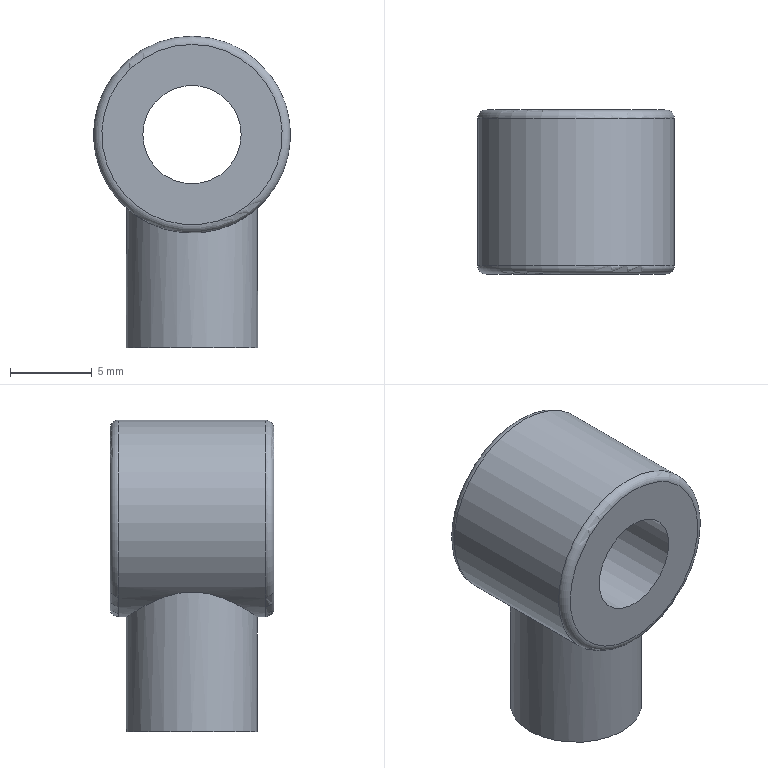Component | NX | PISTON_LINK | 1 solid | 10 faces | box 12 x 10 x 19 mm | volume 1057 mm3 | cylinder 4 | plane 4 | torus 2 | commonest cylinder face diameters 12 x1 6 x1 8 x1 5 x1
STEP:
#1=CARTESIAN_POINT('',(0.,0.,0.));
#2=DIRECTION('',(0.,0.,1.));
#3=DIRECTION('',(1.,0.,0.));
#4=AXIS2_PLACEMENT_3D('',#1,#2,#3);
#5=CARTESIAN_POINT('',(0.,-41.5,133.));
#6=VERTEX_POINT('',#5);
#7=CARTESIAN_POINT('',(0.,-41.5,127.));
#8=DIRECTION('',(0.,1.,0.));
#9=DIRECTION('',(0.,0.,1.));
#10=AXIS2_PLACEMENT_3D('',#7,#8,#9);
#11=CIRCLE('',#10,6.);
#12=CARTESIAN_POINT('',(0.,-32.,127.));
#13=DIRECTION('',(0.,-1.,0.));
#14=DIRECTION('',(0.,0.,1.));
#15=AXIS2_PLACEMENT_3D('',#12,#13,#14);
#16=CYLINDRICAL_SURFACE('',#15,6.);
#17=CARTESIAN_POINT('',(6.283,9.5));
#18=DIRECTION('',(-1.,0.));
#19=VECTOR('',#18,1.);
#20=LINE('',#17,#19);
#21=(GEOMETRIC_REPRESENTATION_CONTEXT(2)PARAMETRIC_REPRESENTATION_CONTEXT()REPRESENTATION_CONTEXT('',''));
#22=DEFINITIONAL_REPRESENTATION('',(#20),#21);
#23=PCURVE('',#16,#22);
#24=CARTESIAN_POINT('',(0.,-41.5,127.));
#25=DIRECTION('',(0.,-1.,0.));
#26=DIRECTION('',(0.,0.,1.));
#27=AXIS2_PLACEMENT_3D('',#24,#25,#26);
#28=TOROIDAL_SURFACE('',#27,5.5,0.5);
#29=CARTESIAN_POINT('',(6.283,6.283));
#30=DIRECTION('',(-1.,0.));
#31=VECTOR('',#30,1.);
#32=LINE('',#29,#31);
#33=(GEOMETRIC_REPRESENTATION_CONTEXT(2)PARAMETRIC_REPRESENTATION_CONTEXT()REPRESENTATION_CONTEXT('',''));
#34=DEFINITIONAL_REPRESENTATION('',(#32),#33);
#35=PCURVE('',#28,#34);
#36=SURFACE_CURVE('',#11,(#23,#35),.PCURVE_S1.);
#37=EDGE_CURVE('',#6,#6,#36,.T.);
#38=ORIENTED_EDGE('',*,*,#37,.T.);
#39=CARTESIAN_POINT('',(0.,-32.5,133.));
#40=VERTEX_POINT('',#39);
#41=CARTESIAN_POINT('',(0.,-32.5,133.));
#42=CARTESIAN_POINT('',(0.,-41.5,133.));
#43=B_SPLINE_CURVE_WITH_KNOTS('',1,(#41,#42),.UNSPECIFIED.,.F.,.F.,(2,2),(0.5,9.5),.PIECEWISE_BEZIER_KNOTS.);
#44=CARTESIAN_POINT('',(0.,0.));
#45=DIRECTION('',(0.,1.));
#46=VECTOR('',#45,1.);
#47=LINE('',#44,#46);
#48=(GEOMETRIC_REPRESENTATION_CONTEXT(2)PARAMETRIC_REPRESENTATION_CONTEXT()REPRESENTATION_CONTEXT('',''));
#49=DEFINITIONAL_REPRESENTATION('',(#47),#48);
#50=PCURVE('',#16,#49);
#51=CARTESIAN_POINT('',(6.283,0.));
#52=DIRECTION('',(0.,1.));
#53=VECTOR('',#52,1.);
#54=LINE('',#51,#53);
#55=(GEOMETRIC_REPRESENTATION_CONTEXT(2)PARAMETRIC_REPRESENTATION_CONTEXT()REPRESENTATION_CONTEXT('',''));
#56=DEFINITIONAL_REPRESENTATION('',(#54),#55);
#57=PCURVE('',#16,#56);
#58=SEAM_CURVE('',#43,(#50,#57),.PCURVE_S1.);
#59=EDGE_CURVE('',#40,#6,#58,.T.);
#60=ORIENTED_EDGE('',*,*,#59,.F.);
#61=CARTESIAN_POINT('',(0.,-32.5,127.));
#62=DIRECTION('',(0.,-1.,0.));
#63=DIRECTION('',(0.,0.,1.));
#64=AXIS2_PLACEMENT_3D('',#61,#62,#63);
#65=CIRCLE('',#64,6.);
#66=CARTESIAN_POINT('',(0.,0.5));
#67=DIRECTION('',(1.,0.));
#68=VECTOR('',#67,1.);
#69=LINE('',#66,#68);
#70=(GEOMETRIC_REPRESENTATION_CONTEXT(2)PARAMETRIC_REPRESENTATION_CONTEXT()REPRESENTATION_CONTEXT('',''));
#71=DEFINITIONAL_REPRESENTATION('',(#69),#70);
#72=PCURVE('',#16,#71);
#73=CARTESIAN_POINT('',(0.,-32.5,127.));
#74=DIRECTION('',(0.,-1.,0.));
#75=DIRECTION('',(0.,0.,1.));
#76=AXIS2_PLACEMENT_3D('',#73,#74,#75);
#77=TOROIDAL_SURFACE('',#76,5.5,0.5);
#78=CARTESIAN_POINT('',(0.,6.283));
#79=DIRECTION('',(1.,0.));
#80=VECTOR('',#79,1.);
#81=LINE('',#78,#80);
#82=(GEOMETRIC_REPRESENTATION_CONTEXT(2)PARAMETRIC_REPRESENTATION_CONTEXT()REPRESENTATION_CONTEXT('',''));
#83=DEFINITIONAL_REPRESENTATION('',(#81),#82);
#84=PCURVE('',#77,#83);
#85=SURFACE_CURVE('',#65,(#72,#84),.PCURVE_S1.);
#86=EDGE_CURVE('',#40,#40,#85,.T.);
#87=ORIENTED_EDGE('',*,*,#86,.T.);
#88=ORIENTED_EDGE('',*,*,#59,.T.);
#89=EDGE_LOOP('',(#38,#60,#87,#88));
#90=FACE_BOUND('',#89,.T.);
#91=CARTESIAN_POINT('',(0.,-33.,121.));
#92=VERTEX_POINT('',#91);
#93=CARTESIAN_POINT('',(1.094,-33.,121.));
#94=CARTESIAN_POINT('',(-1.094,-33.,121.));
#95=CARTESIAN_POINT('',(-2.121,-33.461,121.329));
#96=CARTESIAN_POINT('',(-3.548,-34.894,122.094));
#97=CARTESIAN_POINT('',(-3.998,-35.907,122.526));
#98=CARTESIAN_POINT('',(-4.002,-38.077,122.53));
#99=CARTESIAN_POINT('',(-3.557,-39.094,122.1));
#100=CARTESIAN_POINT('',(-2.124,-40.539,121.33));
#101=CARTESIAN_POINT('',(-1.087,-40.998,121.002));
#102=CARTESIAN_POINT('',(1.069,-41.002,120.998));
#103=CARTESIAN_POINT('',(2.12,-40.54,121.329));
#104=CARTESIAN_POINT('',(3.55,-39.103,122.095));
#105=CARTESIAN_POINT('',(4.,-38.095,122.527));
#106=CARTESIAN_POINT('',(4.,-35.908,122.528));
#107=CARTESIAN_POINT('',(3.55,-34.897,122.095));
#108=CARTESIAN_POINT('',(2.122,-33.462,121.33));
#109=CARTESIAN_POINT('',(1.094,-33.,121.));
#110=CARTESIAN_POINT('',(-1.094,-33.,121.));
#111=B_SPLINE_CURVE_WITH_KNOTS('',3,(#93,#94,#95,#96,#97,#98,#99,#100,#101,#102,#103,#104,#105,#106,#107,#108,#109,#110),.UNSPECIFIED.,.T.,.F.,(2,2,2,2,2,2,2,2,2,2,2),(-0.125,0.,0.125,0.25,0.375,0.5,0.625,0.75,0.875,1.,1.125),.UNSPECIFIED.);
#112=CARTESIAN_POINT('',(3.142,1.));
#113=CARTESIAN_POINT('',(3.108,1.));
#114=CARTESIAN_POINT('',(3.043,1.03));
#115=CARTESIAN_POINT('',(2.947,1.16));
#116=CARTESIAN_POINT('',(2.855,1.367));
#117=CARTESIAN_POINT('',(2.767,1.642));
#118=CARTESIAN_POINT('',(2.686,1.98));
#119=CARTESIAN_POINT('',(2.612,2.371));
#120=CARTESIAN_POINT('',(2.546,2.818));
#121=CARTESIAN_POINT('',(2.491,3.311));
#122=CARTESIAN_POINT('',(2.447,3.843));
#123=CARTESIAN_POINT('',(2.419,4.405));
#124=CARTESIAN_POINT('',(2.408,4.992));
#125=CARTESIAN_POINT('',(2.418,5.58));
#126=CARTESIAN_POINT('',(2.446,6.143));
#127=CARTESIAN_POINT('',(2.489,6.676));
#128=CARTESIAN_POINT('',(2.545,7.172));
#129=CARTESIAN_POINT('',(2.611,7.621));
#130=CARTESIAN_POINT('',(2.685,8.016));
#131=CARTESIAN_POINT('',(2.767,8.355));
#132=CARTESIAN_POINT('',(2.855,8.632));
#133=CARTESIAN_POINT('',(2.947,8.838));
#134=CARTESIAN_POINT('',(3.043,8.969));
#135=CARTESIAN_POINT('',(3.14,9.015));
#136=CARTESIAN_POINT('',(3.238,8.971));
#137=CARTESIAN_POINT('',(3.334,8.841));
#138=CARTESIAN_POINT('',(3.427,8.635));
#139=CARTESIAN_POINT('',(3.515,8.358));
#140=CARTESIAN_POINT('',(3.597,8.02));
#141=CARTESIAN_POINT('',(3.671,7.628));
#142=CARTESIAN_POINT('',(3.737,7.181));
#143=CARTESIAN_POINT('',(3.793,6.688));
#144=CARTESIAN_POINT('',(3.836,6.156));
#145=CARTESIAN_POINT('',(3.864,5.593));
#146=CARTESIAN_POINT('',(3.875,5.002));
#147=CARTESIAN_POINT('',(3.864,4.41));
#148=CARTESIAN_POINT('',(3.836,3.846));
#149=CARTESIAN_POINT('',(3.793,3.313));
#150=CARTESIAN_POINT('',(3.737,2.82));
#151=CARTESIAN_POINT('',(3.671,2.373));
#152=CARTESIAN_POINT('',(3.597,1.981));
#153=CARTESIAN_POINT('',(3.516,1.643));
#154=CARTESIAN_POINT('',(3.428,1.367));
#155=CARTESIAN_POINT('',(3.336,1.16));
#156=CARTESIAN_POINT('',(3.24,1.031));
#157=CARTESIAN_POINT('',(3.175,1.));
#158=CARTESIAN_POINT('',(3.142,1.));
#159=B_SPLINE_CURVE_WITH_KNOTS('',3,(#112,#113,#114,#115,#116,#117,#118,#119,#120,#121,#122,#123,#124,#125,#126,#127,#128,#129,#130,#131,#132,#133,#134,#135,#136,#137,#138,#139,#140,#141,#142,#143,#144,#145,#146,#147,#148,#149,#150,#151,#152,#153,#154,#155,#156,#157,#158),.UNSPECIFIED.,.T.,.F.,(4,1,1,1,1,1,1,1,1,1,1,1,1,1,1,1,1,1,1,1,1,1,1,1,1,1,1,1,1,1,1,1,1,1,1,1,1,1,1,1,1,1,1,1,4),(0.,0.02273,0.04545,0.06818,0.09091,0.1136,0.1364,0.1591,0.1818,0.2045,0.2273,0.25,0.2727,0.2955,0.3182,0.3409,0.3636,0.3864,0.4091,0.4318,0.4545,0.4773,0.5,0.5227,0.5455,0.5682,0.5909,0.6136,0.6364,0.6591,0.6818,0.7045,0.7273,0.75,0.7727,0.7955,0.8182,0.8409,0.8636,0.8864,0.9091,0.9318,0.9545,0.9773,1.),.QUASI_UNIFORM_KNOTS.);
#160=(GEOMETRIC_REPRESENTATION_CONTEXT(2)PARAMETRIC_REPRESENTATION_CONTEXT()REPRESENTATION_CONTEXT('',''));
#161=DEFINITIONAL_REPRESENTATION('',(#159),#160);
#162=PCURVE('',#16,#161);
#163=CARTESIAN_POINT('',(0.,-37.,114.));
#164=DIRECTION('',(0.,0.,1.));
#165=DIRECTION('',(0.,1.,0.));
#166=AXIS2_PLACEMENT_3D('',#163,#164,#165);
#167=CYLINDRICAL_SURFACE('',#166,4.);
#168=CARTESIAN_POINT('',(0.,7.));
#169=CARTESIAN_POINT('',(0.04968,7.));
#170=CARTESIAN_POINT('',(0.1481,7.022));
#171=CARTESIAN_POINT('',(0.2934,7.11));
#172=CARTESIAN_POINT('',(0.437,7.243));
#173=CARTESIAN_POINT('',(0.5788,7.412));
#174=CARTESIAN_POINT('',(0.7187,7.606));
#175=CARTESIAN_POINT('',(0.8564,7.817));
#176=CARTESIAN_POINT('',(0.9956,8.029));
#177=CARTESIAN_POINT('',(1.136,8.224));
#178=CARTESIAN_POINT('',(1.278,8.387));
#179=CARTESIAN_POINT('',(1.422,8.498));
#180=CARTESIAN_POINT('',(1.569,8.542));
#181=CARTESIAN_POINT('',(1.716,8.5));
#182=CARTESIAN_POINT('',(1.86,8.39));
#183=CARTESIAN_POINT('',(2.002,8.229));
#184=CARTESIAN_POINT('',(2.143,8.033));
#185=CARTESIAN_POINT('',(2.283,7.821));
#186=CARTESIAN_POINT('',(2.421,7.609));
#187=CARTESIAN_POINT('',(2.562,7.414));
#188=CARTESIAN_POINT('',(2.704,7.244));
#189=CARTESIAN_POINT('',(2.848,7.111));
#190=CARTESIAN_POINT('',(2.993,7.022));
#191=CARTESIAN_POINT('',(3.139,6.989));
#192=CARTESIAN_POINT('',(3.286,7.021));
#193=CARTESIAN_POINT('',(3.432,7.109));
#194=CARTESIAN_POINT('',(3.576,7.242));
#195=CARTESIAN_POINT('',(3.719,7.412));
#196=CARTESIAN_POINT('',(3.86,7.606));
#197=CARTESIAN_POINT('',(3.998,7.817));
#198=CARTESIAN_POINT('',(4.138,8.03));
#199=CARTESIAN_POINT('',(4.278,8.225));
#200=CARTESIAN_POINT('',(4.42,8.388));
#201=CARTESIAN_POINT('',(4.564,8.499));
#202=CARTESIAN_POINT('',(4.712,8.542));
#203=CARTESIAN_POINT('',(4.86,8.499));
#204=CARTESIAN_POINT('',(5.004,8.388));
#205=CARTESIAN_POINT('',(5.146,8.226));
#206=CARTESIAN_POINT('',(5.287,8.03));
#207=CARTESIAN_POINT('',(5.426,7.818));
#208=CARTESIAN_POINT('',(5.564,7.607));
#209=CARTESIAN_POINT('',(5.704,7.413));
#210=CARTESIAN_POINT('',(5.846,7.243));
#211=CARTESIAN_POINT('',(5.99,7.11));
#212=CARTESIAN_POINT('',(6.135,7.022));
#213=CARTESIAN_POINT('',(6.234,7.));
#214=CARTESIAN_POINT('',(6.283,7.));
#215=B_SPLINE_CURVE_WITH_KNOTS('',3,(#168,#169,#170,#171,#172,#173,#174,#175,#176,#177,#178,#179,#180,#181,#182,#183,#184,#185,#186,#187,#188,#189,#190,#191,#192,#193,#194,#195,#196,#197,#198,#199,#200,#201,#202,#203,#204,#205,#206,#207,#208,#209,#210,#211,#212,#213,#214),.UNSPECIFIED.,.F.,.F.,(4,1,1,1,1,1,1,1,1,1,1,1,1,1,1,1,1,1,1,1,1,1,1,1,1,1,1,1,1,1,1,1,1,1,1,1,1,1,1,1,1,1,1,1,4),(0.,0.02273,0.04545,0.06818,0.09091,0.1136,0.1364,0.1591,0.1818,0.2045,0.2273,0.25,0.2727,0.2955,0.3182,0.3409,0.3636,0.3864,0.4091,0.4318,0.4545,0.4773,0.5,0.5227,0.5455,0.5682,0.5909,0.6136,0.6364,0.6591,0.6818,0.7045,0.7273,0.75,0.7727,0.7955,0.8182,0.8409,0.8636,0.8864,0.9091,0.9318,0.9545,0.9773,1.),.QUASI_UNIFORM_KNOTS.);
#216=(GEOMETRIC_REPRESENTATION_CONTEXT(2)PARAMETRIC_REPRESENTATION_CONTEXT()REPRESENTATION_CONTEXT('',''));
#217=DEFINITIONAL_REPRESENTATION('',(#215),#216);
#218=PCURVE('',#167,#217);
#219=SURFACE_CURVE('',#111,(#162,#218),.PCURVE_S1.);
#220=EDGE_CURVE('',#92,#92,#219,.T.);
#221=ORIENTED_EDGE('',*,*,#220,.T.);
#222=EDGE_LOOP('',(#221));
#223=FACE_BOUND('',#222,.T.);
#224=ADVANCED_FACE('',(#90,#223),#16,.T.);
#225=CARTESIAN_POINT('',(-3.,-32.,127.));
#226=VERTEX_POINT('',#225);
#227=CARTESIAN_POINT('',(0.,-32.,127.));
#228=DIRECTION('',(0.,-1.,0.));
#229=DIRECTION('',(-1.,0.,0.));
#230=AXIS2_PLACEMENT_3D('',#227,#228,#229);
#231=CIRCLE('',#230,3.);
#232=CARTESIAN_POINT('',(0.,-32.,127.));
#233=DIRECTION('',(0.,-1.,0.));
#234=DIRECTION('',(0.,0.,1.));
#235=AXIS2_PLACEMENT_3D('',#232,#233,#234);
#236=CYLINDRICAL_SURFACE('',#235,3.);
#237=CARTESIAN_POINT('',(1.571,0.));
#238=DIRECTION('',(1.,0.));
#239=VECTOR('',#238,1.);
#240=LINE('',#237,#239);
#241=(GEOMETRIC_REPRESENTATION_CONTEXT(2)PARAMETRIC_REPRESENTATION_CONTEXT()REPRESENTATION_CONTEXT('',''));
#242=DEFINITIONAL_REPRESENTATION('',(#240),#241);
#243=PCURVE('',#236,#242);
#244=CARTESIAN_POINT('',(0.,-32.,127.));
#245=DIRECTION('',(0.,-1.,0.));
#246=DIRECTION('',(0.,0.,1.));
#247=AXIS2_PLACEMENT_3D('',#244,#245,#246);
#248=PLANE('',#247);
#249=CARTESIAN_POINT('',(0.,0.));
#250=DIRECTION('',(0.,1.));
#251=AXIS2_PLACEMENT_2D('',#249,#250);
#252=CIRCLE('',#251,3.);
#253=(GEOMETRIC_REPRESENTATION_CONTEXT(2)PARAMETRIC_REPRESENTATION_CONTEXT()REPRESENTATION_CONTEXT('',''));
#254=DEFINITIONAL_REPRESENTATION('',(#252),#253);
#255=PCURVE('',#248,#254);
#256=SURFACE_CURVE('',#231,(#243,#255),.PCURVE_S1.);
#257=EDGE_CURVE('',#226,#226,#256,.T.);
#258=ORIENTED_EDGE('',*,*,#257,.T.);
#259=CARTESIAN_POINT('',(-3.,-42.,127.));
#260=VERTEX_POINT('',#259);
#261=CARTESIAN_POINT('',(-3.,-32.,127.));
#262=CARTESIAN_POINT('',(-3.,-42.,127.));
#263=B_SPLINE_CURVE_WITH_KNOTS('',1,(#261,#262),.UNSPECIFIED.,.F.,.F.,(2,2),(0.,10.),.PIECEWISE_BEZIER_KNOTS.);
#264=CARTESIAN_POINT('',(7.854,0.));
#265=DIRECTION('',(0.,1.));
#266=VECTOR('',#265,1.);
#267=LINE('',#264,#266);
#268=(GEOMETRIC_REPRESENTATION_CONTEXT(2)PARAMETRIC_REPRESENTATION_CONTEXT()REPRESENTATION_CONTEXT('',''));
#269=DEFINITIONAL_REPRESENTATION('',(#267),#268);
#270=PCURVE('',#236,#269);
#271=CARTESIAN_POINT('',(1.571,0.));
#272=DIRECTION('',(0.,1.));
#273=VECTOR('',#272,1.);
#274=LINE('',#271,#273);
#275=(GEOMETRIC_REPRESENTATION_CONTEXT(2)PARAMETRIC_REPRESENTATION_CONTEXT()REPRESENTATION_CONTEXT('',''));
#276=DEFINITIONAL_REPRESENTATION('',(#274),#275);
#277=PCURVE('',#236,#276);
#278=SEAM_CURVE('',#263,(#270,#277),.PCURVE_S1.);
#279=EDGE_CURVE('',#226,#260,#278,.T.);
#280=ORIENTED_EDGE('',*,*,#279,.T.);
#281=CARTESIAN_POINT('',(0.,-42.,127.));
#282=DIRECTION('',(0.,-1.,0.));
#283=DIRECTION('',(-1.,0.,0.));
#284=AXIS2_PLACEMENT_3D('',#281,#282,#283);
#285=CIRCLE('',#284,3.);
#286=CARTESIAN_POINT('',(1.571,10.));
#287=DIRECTION('',(1.,0.));
#288=VECTOR('',#287,1.);
#289=LINE('',#286,#288);
#290=(GEOMETRIC_REPRESENTATION_CONTEXT(2)PARAMETRIC_REPRESENTATION_CONTEXT()REPRESENTATION_CONTEXT('',''));
#291=DEFINITIONAL_REPRESENTATION('',(#289),#290);
#292=PCURVE('',#236,#291);
#293=CARTESIAN_POINT('',(0.,-42.,127.));
#294=DIRECTION('',(0.,-1.,0.));
#295=DIRECTION('',(0.,0.,1.));
#296=AXIS2_PLACEMENT_3D('',#293,#294,#295);
#297=PLANE('',#296);
#298=CARTESIAN_POINT('',(0.,0.));
#299=DIRECTION('',(0.,1.));
#300=AXIS2_PLACEMENT_2D('',#298,#299);
#301=CIRCLE('',#300,3.);
#302=(GEOMETRIC_REPRESENTATION_CONTEXT(2)PARAMETRIC_REPRESENTATION_CONTEXT()REPRESENTATION_CONTEXT('',''));
#303=DEFINITIONAL_REPRESENTATION('',(#301),#302);
#304=PCURVE('',#297,#303);
#305=SURFACE_CURVE('',#285,(#292,#304),.PCURVE_S1.);
#306=EDGE_CURVE('',#260,#260,#305,.T.);
#307=ORIENTED_EDGE('',*,*,#306,.F.);
#308=ORIENTED_EDGE('',*,*,#279,.F.);
#309=EDGE_LOOP('',(#258,#280,#307,#308));
#310=FACE_BOUND('',#309,.F.);
#311=ADVANCED_FACE('',(#310),#236,.F.);
#312=CARTESIAN_POINT('',(0.,-32.,132.5));
#313=VERTEX_POINT('',#312);
#314=CARTESIAN_POINT('',(0.,-32.,127.));
#315=DIRECTION('',(0.,1.,0.));
#316=DIRECTION('',(0.,0.,1.));
#317=AXIS2_PLACEMENT_3D('',#314,#315,#316);
#318=CIRCLE('',#317,5.5);
#319=CARTESIAN_POINT('',(5.5,0.));
#320=CARTESIAN_POINT('',(5.5,-9.526));
#321=CARTESIAN_POINT('',(-2.75,-4.763));
#322=CARTESIAN_POINT('',(-11.,-0.));
#323=CARTESIAN_POINT('',(-2.75,4.763));
#324=CARTESIAN_POINT('',(5.5,9.526));
#325=CARTESIAN_POINT('',(5.5,0.));
#326=(BOUNDED_CURVE()B_SPLINE_CURVE(2,(#319,#320,#321,#322,#323,#324,#325),.UNSPECIFIED.,.T.,.F.)B_SPLINE_CURVE_WITH_KNOTS((1,2,2,2,2,1),(-2.094,0.,2.094,4.189,6.283,8.378),.UNSPECIFIED.)CURVE()GEOMETRIC_REPRESENTATION_ITEM()RATIONAL_B_SPLINE_CURVE((1.,0.5,1.,0.5,1.,0.5,1.))REPRESENTATION_ITEM(''));
#327=(GEOMETRIC_REPRESENTATION_CONTEXT(2)PARAMETRIC_REPRESENTATION_CONTEXT()REPRESENTATION_CONTEXT('',''));
#328=DEFINITIONAL_REPRESENTATION('',(#326),#327);
#329=PCURVE('',#248,#328);
#330=CARTESIAN_POINT('',(6.283,4.712));
#331=DIRECTION('',(-1.,0.));
#332=VECTOR('',#331,1.);
#333=LINE('',#330,#332);
#334=(GEOMETRIC_REPRESENTATION_CONTEXT(2)PARAMETRIC_REPRESENTATION_CONTEXT()REPRESENTATION_CONTEXT('',''));
#335=DEFINITIONAL_REPRESENTATION('',(#333),#334);
#336=PCURVE('',#77,#335);
#337=SURFACE_CURVE('',#318,(#329,#336),.PCURVE_S1.);
#338=EDGE_CURVE('',#313,#313,#337,.T.);
#339=ORIENTED_EDGE('',*,*,#338,.T.);
#340=EDGE_LOOP('',(#339));
#341=FACE_BOUND('',#340,.T.);
#342=ORIENTED_EDGE('',*,*,#257,.T.);
#343=EDGE_LOOP('',(#342));
#344=FACE_BOUND('',#343,.T.);
#345=ADVANCED_FACE('',(#341,#344),#248,.F.);
#346=CARTESIAN_POINT('',(0.,-42.,132.5));
#347=VERTEX_POINT('',#346);
#348=CARTESIAN_POINT('',(0.,-42.,127.));
#349=DIRECTION('',(0.,-1.,0.));
#350=DIRECTION('',(0.,0.,1.));
#351=AXIS2_PLACEMENT_3D('',#348,#349,#350);
#352=CIRCLE('',#351,5.5);
#353=CARTESIAN_POINT('',(0.,0.));
#354=DIRECTION('',(1.,0.));
#355=AXIS2_PLACEMENT_2D('',#353,#354);
#356=CIRCLE('',#355,5.5);
#357=(GEOMETRIC_REPRESENTATION_CONTEXT(2)PARAMETRIC_REPRESENTATION_CONTEXT()REPRESENTATION_CONTEXT('',''));
#358=DEFINITIONAL_REPRESENTATION('',(#356),#357);
#359=PCURVE('',#297,#358);
#360=CARTESIAN_POINT('',(0.,7.854));
#361=DIRECTION('',(1.,0.));
#362=VECTOR('',#361,1.);
#363=LINE('',#360,#362);
#364=(GEOMETRIC_REPRESENTATION_CONTEXT(2)PARAMETRIC_REPRESENTATION_CONTEXT()REPRESENTATION_CONTEXT('',''));
#365=DEFINITIONAL_REPRESENTATION('',(#363),#364);
#366=PCURVE('',#28,#365);
#367=SURFACE_CURVE('',#352,(#359,#366),.PCURVE_S1.);
#368=EDGE_CURVE('',#347,#347,#367,.T.);
#369=ORIENTED_EDGE('',*,*,#368,.T.);
#370=EDGE_LOOP('',(#369));
#371=FACE_BOUND('',#370,.T.);
#372=ORIENTED_EDGE('',*,*,#306,.F.);
#373=EDGE_LOOP('',(#372));
#374=FACE_BOUND('',#373,.T.);
#375=ADVANCED_FACE('',(#371,#374),#297,.T.);
#376=ORIENTED_EDGE('',*,*,#220,.F.);
#377=CARTESIAN_POINT('',(0.,-33.,114.));
#378=VERTEX_POINT('',#377);
#379=CARTESIAN_POINT('',(0.,-33.,114.));
#380=CARTESIAN_POINT('',(0.,-33.,121.));
#381=B_SPLINE_CURVE_WITH_KNOTS('',1,(#379,#380),.UNSPECIFIED.,.F.,.F.,(2,2),(0.,7.),.PIECEWISE_BEZIER_KNOTS.);
#382=CARTESIAN_POINT('',(0.,0.));
#383=DIRECTION('',(0.,1.));
#384=VECTOR('',#383,1.);
#385=LINE('',#382,#384);
#386=(GEOMETRIC_REPRESENTATION_CONTEXT(2)PARAMETRIC_REPRESENTATION_CONTEXT()REPRESENTATION_CONTEXT('',''));
#387=DEFINITIONAL_REPRESENTATION('',(#385),#386);
#388=PCURVE('',#167,#387);
#389=CARTESIAN_POINT('',(6.283,0.));
#390=DIRECTION('',(0.,1.));
#391=VECTOR('',#390,1.);
#392=LINE('',#389,#391);
#393=(GEOMETRIC_REPRESENTATION_CONTEXT(2)PARAMETRIC_REPRESENTATION_CONTEXT()REPRESENTATION_CONTEXT('',''));
#394=DEFINITIONAL_REPRESENTATION('',(#392),#393);
#395=PCURVE('',#167,#394);
#396=SEAM_CURVE('',#381,(#388,#395),.PCURVE_S1.);
#397=EDGE_CURVE('',#378,#92,#396,.T.);
#398=ORIENTED_EDGE('',*,*,#397,.F.);
#399=CARTESIAN_POINT('',(0.,-37.,114.));
#400=DIRECTION('',(0.,0.,-1.));
#401=DIRECTION('',(-0.,1.,0.));
#402=AXIS2_PLACEMENT_3D('',#399,#400,#401);
#403=CIRCLE('',#402,4.);
#404=CARTESIAN_POINT('',(6.283,0.));
#405=DIRECTION('',(-1.,0.));
#406=VECTOR('',#405,1.);
#407=LINE('',#404,#406);
#408=(GEOMETRIC_REPRESENTATION_CONTEXT(2)PARAMETRIC_REPRESENTATION_CONTEXT()REPRESENTATION_CONTEXT('',''));
#409=DEFINITIONAL_REPRESENTATION('',(#407),#408);
#410=PCURVE('',#167,#409);
#411=CARTESIAN_POINT('',(0.,-37.,114.));
#412=DIRECTION('',(0.,0.,-1.));
#413=DIRECTION('',(0.,-1.,0.));
#414=AXIS2_PLACEMENT_3D('',#411,#412,#413);
#415=PLANE('',#414);
#416=CARTESIAN_POINT('',(0.,0.));
#417=DIRECTION('',(-1.,0.));
#418=AXIS2_PLACEMENT_2D('',#416,#417);
#419=CIRCLE('',#418,4.);
#420=(GEOMETRIC_REPRESENTATION_CONTEXT(2)PARAMETRIC_REPRESENTATION_CONTEXT()REPRESENTATION_CONTEXT('',''));
#421=DEFINITIONAL_REPRESENTATION('',(#419),#420);
#422=PCURVE('',#415,#421);
#423=SURFACE_CURVE('',#403,(#410,#422),.PCURVE_S1.);
#424=EDGE_CURVE('',#378,#378,#423,.T.);
#425=ORIENTED_EDGE('',*,*,#424,.F.);
#426=ORIENTED_EDGE('',*,*,#397,.T.);
#427=EDGE_LOOP('',(#376,#398,#425,#426));
#428=FACE_BOUND('',#427,.T.);
#429=ADVANCED_FACE('',(#428),#167,.T.);
#430=CARTESIAN_POINT('',(0.,-34.5,114.));
#431=VERTEX_POINT('',#430);
#432=CARTESIAN_POINT('',(0.,-37.,114.));
#433=DIRECTION('',(0.,0.,1.));
#434=DIRECTION('',(0.,1.,0.));
#435=AXIS2_PLACEMENT_3D('',#432,#433,#434);
#436=CIRCLE('',#435,2.5);
#437=CARTESIAN_POINT('',(-2.5,0.));
#438=CARTESIAN_POINT('',(-2.5,4.33));
#439=CARTESIAN_POINT('',(1.25,2.165));
#440=CARTESIAN_POINT('',(5.,0.));
#441=CARTESIAN_POINT('',(1.25,-2.165));
#442=CARTESIAN_POINT('',(-2.5,-4.33));
#443=CARTESIAN_POINT('',(-2.5,0.));
#444=(BOUNDED_CURVE()B_SPLINE_CURVE(2,(#437,#438,#439,#440,#441,#442,#443),.UNSPECIFIED.,.T.,.F.)B_SPLINE_CURVE_WITH_KNOTS((1,2,2,2,2,1),(-2.094,0.,2.094,4.189,6.283,8.378),.UNSPECIFIED.)CURVE()GEOMETRIC_REPRESENTATION_ITEM()RATIONAL_B_SPLINE_CURVE((1.,0.5,1.,0.5,1.,0.5,1.))REPRESENTATION_ITEM(''));
#445=(GEOMETRIC_REPRESENTATION_CONTEXT(2)PARAMETRIC_REPRESENTATION_CONTEXT()REPRESENTATION_CONTEXT('',''));
#446=DEFINITIONAL_REPRESENTATION('',(#444),#445);
#447=PCURVE('',#415,#446);
#448=CARTESIAN_POINT('',(0.,-37.,122.));
#449=DIRECTION('',(0.,0.,-1.));
#450=DIRECTION('',(0.,-1.,0.));
#451=AXIS2_PLACEMENT_3D('',#448,#449,#450);
#452=CYLINDRICAL_SURFACE('',#451,2.5);
#453=CARTESIAN_POINT('',(9.425,8.));
#454=DIRECTION('',(-1.,0.));
#455=VECTOR('',#454,1.);
#456=LINE('',#453,#455);
#457=(GEOMETRIC_REPRESENTATION_CONTEXT(2)PARAMETRIC_REPRESENTATION_CONTEXT()REPRESENTATION_CONTEXT('',''));
#458=DEFINITIONAL_REPRESENTATION('',(#456),#457);
#459=PCURVE('',#452,#458);
#460=SURFACE_CURVE('',#436,(#447,#459),.PCURVE_S1.);
#461=EDGE_CURVE('',#431,#431,#460,.T.);
#462=ORIENTED_EDGE('',*,*,#461,.T.);
#463=EDGE_LOOP('',(#462));
#464=FACE_BOUND('',#463,.T.);
#465=ORIENTED_EDGE('',*,*,#424,.T.);
#466=EDGE_LOOP('',(#465));
#467=FACE_BOUND('',#466,.T.);
#468=ADVANCED_FACE('',(#464,#467),#415,.T.);
#469=CARTESIAN_POINT('',(0.,-34.5,122.));
#470=VERTEX_POINT('',#469);
#471=CARTESIAN_POINT('',(0.,-37.,122.));
#472=DIRECTION('',(0.,0.,-1.));
#473=DIRECTION('',(0.,1.,0.));
#474=AXIS2_PLACEMENT_3D('',#471,#472,#473);
#475=CIRCLE('',#474,2.5);
#476=CARTESIAN_POINT('',(3.142,0.));
#477=DIRECTION('',(1.,0.));
#478=VECTOR('',#477,1.);
#479=LINE('',#476,#478);
#480=(GEOMETRIC_REPRESENTATION_CONTEXT(2)PARAMETRIC_REPRESENTATION_CONTEXT()REPRESENTATION_CONTEXT('',''));
#481=DEFINITIONAL_REPRESENTATION('',(#479),#480);
#482=PCURVE('',#452,#481);
#483=CARTESIAN_POINT('',(0.,-37.,122.));
#484=DIRECTION('',(0.,0.,1.));
#485=DIRECTION('',(0.,1.,0.));
#486=AXIS2_PLACEMENT_3D('',#483,#484,#485);
#487=PLANE('',#486);
#488=CARTESIAN_POINT('',(2.5,0.));
#489=CARTESIAN_POINT('',(2.5,-4.33));
#490=CARTESIAN_POINT('',(-1.25,-2.165));
#491=CARTESIAN_POINT('',(-5.,-0.));
#492=CARTESIAN_POINT('',(-1.25,2.165));
#493=CARTESIAN_POINT('',(2.5,4.33));
#494=CARTESIAN_POINT('',(2.5,0.));
#495=(BOUNDED_CURVE()B_SPLINE_CURVE(2,(#488,#489,#490,#491,#492,#493,#494),.UNSPECIFIED.,.T.,.F.)B_SPLINE_CURVE_WITH_KNOTS((1,2,2,2,2,1),(-2.094,0.,2.094,4.189,6.283,8.378),.UNSPECIFIED.)CURVE()GEOMETRIC_REPRESENTATION_ITEM()RATIONAL_B_SPLINE_CURVE((1.,0.5,1.,0.5,1.,0.5,1.))REPRESENTATION_ITEM(''));
#496=(GEOMETRIC_REPRESENTATION_CONTEXT(2)PARAMETRIC_REPRESENTATION_CONTEXT()REPRESENTATION_CONTEXT('',''));
#497=DEFINITIONAL_REPRESENTATION('',(#495),#496);
#498=PCURVE('',#487,#497);
#499=SURFACE_CURVE('',#475,(#482,#498),.PCURVE_S1.);
#500=EDGE_CURVE('',#470,#470,#499,.T.);
#501=ORIENTED_EDGE('',*,*,#500,.T.);
#502=CARTESIAN_POINT('',(0.,-34.5,122.));
#503=CARTESIAN_POINT('',(0.,-34.5,114.));
#504=B_SPLINE_CURVE_WITH_KNOTS('',1,(#502,#503),.UNSPECIFIED.,.F.,.F.,(2,2),(0.,8.),.PIECEWISE_BEZIER_KNOTS.);
#505=CARTESIAN_POINT('',(9.425,0.));
#506=DIRECTION('',(0.,1.));
#507=VECTOR('',#506,1.);
#508=LINE('',#505,#507);
#509=(GEOMETRIC_REPRESENTATION_CONTEXT(2)PARAMETRIC_REPRESENTATION_CONTEXT()REPRESENTATION_CONTEXT('',''));
#510=DEFINITIONAL_REPRESENTATION('',(#508),#509);
#511=PCURVE('',#452,#510);
#512=CARTESIAN_POINT('',(3.142,0.));
#513=DIRECTION('',(0.,1.));
#514=VECTOR('',#513,1.);
#515=LINE('',#512,#514);
#516=(GEOMETRIC_REPRESENTATION_CONTEXT(2)PARAMETRIC_REPRESENTATION_CONTEXT()REPRESENTATION_CONTEXT('',''));
#517=DEFINITIONAL_REPRESENTATION('',(#515),#516);
#518=PCURVE('',#452,#517);
#519=SEAM_CURVE('',#504,(#511,#518),.PCURVE_S1.);
#520=EDGE_CURVE('',#470,#431,#519,.T.);
#521=ORIENTED_EDGE('',*,*,#520,.T.);
#522=ORIENTED_EDGE('',*,*,#461,.T.);
#523=ORIENTED_EDGE('',*,*,#520,.F.);
#524=EDGE_LOOP('',(#501,#521,#522,#523));
#525=FACE_BOUND('',#524,.F.);
#526=ADVANCED_FACE('',(#525),#452,.F.);
#527=ORIENTED_EDGE('',*,*,#500,.T.);
#528=EDGE_LOOP('',(#527));
#529=FACE_BOUND('',#528,.T.);
#530=ADVANCED_FACE('',(#529),#487,.F.);
#531=ORIENTED_EDGE('',*,*,#37,.F.);
#532=CARTESIAN_POINT('',(0.,-41.5,133.));
#533=CARTESIAN_POINT('',(0.,-41.634,133.));
#534=CARTESIAN_POINT('',(0.,-41.764,132.957));
#535=CARTESIAN_POINT('',(0.,-41.876,132.876));
#536=CARTESIAN_POINT('',(0.,-41.957,132.764));
#537=CARTESIAN_POINT('',(0.,-42.,132.634));
#538=CARTESIAN_POINT('',(0.,-42.,132.5));
#539=(BOUNDED_CURVE()B_SPLINE_CURVE(6,(#532,#533,#534,#535,#536,#537,#538),.UNSPECIFIED.,.F.,.F.)B_SPLINE_CURVE_WITH_KNOTS((7,7),(0.,1.571),.PIECEWISE_BEZIER_KNOTS.)CURVE()GEOMETRIC_REPRESENTATION_ITEM()RATIONAL_B_SPLINE_CURVE((1.031,1.01,0.9979,0.994,0.9979,1.01,1.031))REPRESENTATION_ITEM(''));
#540=CARTESIAN_POINT('',(6.283,6.283));
#541=DIRECTION('',(0.,1.));
#542=VECTOR('',#541,1.);
#543=LINE('',#540,#542);
#544=(GEOMETRIC_REPRESENTATION_CONTEXT(2)PARAMETRIC_REPRESENTATION_CONTEXT()REPRESENTATION_CONTEXT('',''));
#545=DEFINITIONAL_REPRESENTATION('',(#543),#544);
#546=PCURVE('',#28,#545);
#547=CARTESIAN_POINT('',(0.,6.283));
#548=DIRECTION('',(0.,1.));
#549=VECTOR('',#548,1.);
#550=LINE('',#547,#549);
#551=(GEOMETRIC_REPRESENTATION_CONTEXT(2)PARAMETRIC_REPRESENTATION_CONTEXT()REPRESENTATION_CONTEXT('',''));
#552=DEFINITIONAL_REPRESENTATION('',(#550),#551);
#553=PCURVE('',#28,#552);
#554=SEAM_CURVE('',#539,(#546,#553),.PCURVE_S1.);
#555=EDGE_CURVE('',#6,#347,#554,.T.);
#556=ORIENTED_EDGE('',*,*,#555,.T.);
#557=ORIENTED_EDGE('',*,*,#368,.F.);
#558=ORIENTED_EDGE('',*,*,#555,.F.);
#559=EDGE_LOOP('',(#531,#556,#557,#558));
#560=FACE_BOUND('',#559,.T.);
#561=ADVANCED_FACE('',(#560),#28,.T.);
#562=ORIENTED_EDGE('',*,*,#338,.F.);
#563=CARTESIAN_POINT('',(0.,-32.,132.5));
#564=CARTESIAN_POINT('',(0.,-32.,132.634));
#565=CARTESIAN_POINT('',(0.,-32.043,132.764));
#566=CARTESIAN_POINT('',(0.,-32.124,132.876));
#567=CARTESIAN_POINT('',(0.,-32.236,132.957));
#568=CARTESIAN_POINT('',(0.,-32.366,133.));
#569=CARTESIAN_POINT('',(0.,-32.5,133.));
#570=(BOUNDED_CURVE()B_SPLINE_CURVE(6,(#563,#564,#565,#566,#567,#568,#569),.UNSPECIFIED.,.F.,.F.)B_SPLINE_CURVE_WITH_KNOTS((7,7),(4.712,6.283),.PIECEWISE_BEZIER_KNOTS.)CURVE()GEOMETRIC_REPRESENTATION_ITEM()RATIONAL_B_SPLINE_CURVE((1.031,1.01,0.9979,0.994,0.9979,1.01,1.031))REPRESENTATION_ITEM(''));
#571=CARTESIAN_POINT('',(6.283,0.));
#572=DIRECTION('',(0.,1.));
#573=VECTOR('',#572,1.);
#574=LINE('',#571,#573);
#575=(GEOMETRIC_REPRESENTATION_CONTEXT(2)PARAMETRIC_REPRESENTATION_CONTEXT()REPRESENTATION_CONTEXT('',''));
#576=DEFINITIONAL_REPRESENTATION('',(#574),#575);
#577=PCURVE('',#77,#576);
#578=CARTESIAN_POINT('',(0.,0.));
#579=DIRECTION('',(0.,1.));
#580=VECTOR('',#579,1.);
#581=LINE('',#578,#580);
#582=(GEOMETRIC_REPRESENTATION_CONTEXT(2)PARAMETRIC_REPRESENTATION_CONTEXT()REPRESENTATION_CONTEXT('',''));
#583=DEFINITIONAL_REPRESENTATION('',(#581),#582);
#584=PCURVE('',#77,#583);
#585=SEAM_CURVE('',#570,(#577,#584),.PCURVE_S1.);
#586=EDGE_CURVE('',#313,#40,#585,.T.);
#587=ORIENTED_EDGE('',*,*,#586,.T.);
#588=ORIENTED_EDGE('',*,*,#86,.F.);
#589=ORIENTED_EDGE('',*,*,#586,.F.);
#590=EDGE_LOOP('',(#562,#587,#588,#589));
#591=FACE_BOUND('',#590,.T.);
#592=ADVANCED_FACE('',(#591),#77,.T.);
#593=CLOSED_SHELL('',(#224,#311,#345,#375,#429,#468,#526,#530,#561,#592));
#594=MANIFOLD_SOLID_BREP('',#593);
#595=(LENGTH_UNIT()NAMED_UNIT(*)SI_UNIT(.MILLI.,.METRE.));
#596=UNCERTAINTY_MEASURE_WITH_UNIT(LENGTH_MEASURE(0.0005),#595,'','');
#597=(NAMED_UNIT(*)PLANE_ANGLE_UNIT()SI_UNIT($,.RADIAN.));
#598=(NAMED_UNIT(*)SI_UNIT($,.STERADIAN.)SOLID_ANGLE_UNIT());
#599=(GEOMETRIC_REPRESENTATION_CONTEXT(3)GLOBAL_UNCERTAINTY_ASSIGNED_CONTEXT((#596))GLOBAL_UNIT_ASSIGNED_CONTEXT((#595,#597,#598))REPRESENTATION_CONTEXT('',''));
#600=ADVANCED_BREP_SHAPE_REPRESENTATION('',(#4,#594),#599);